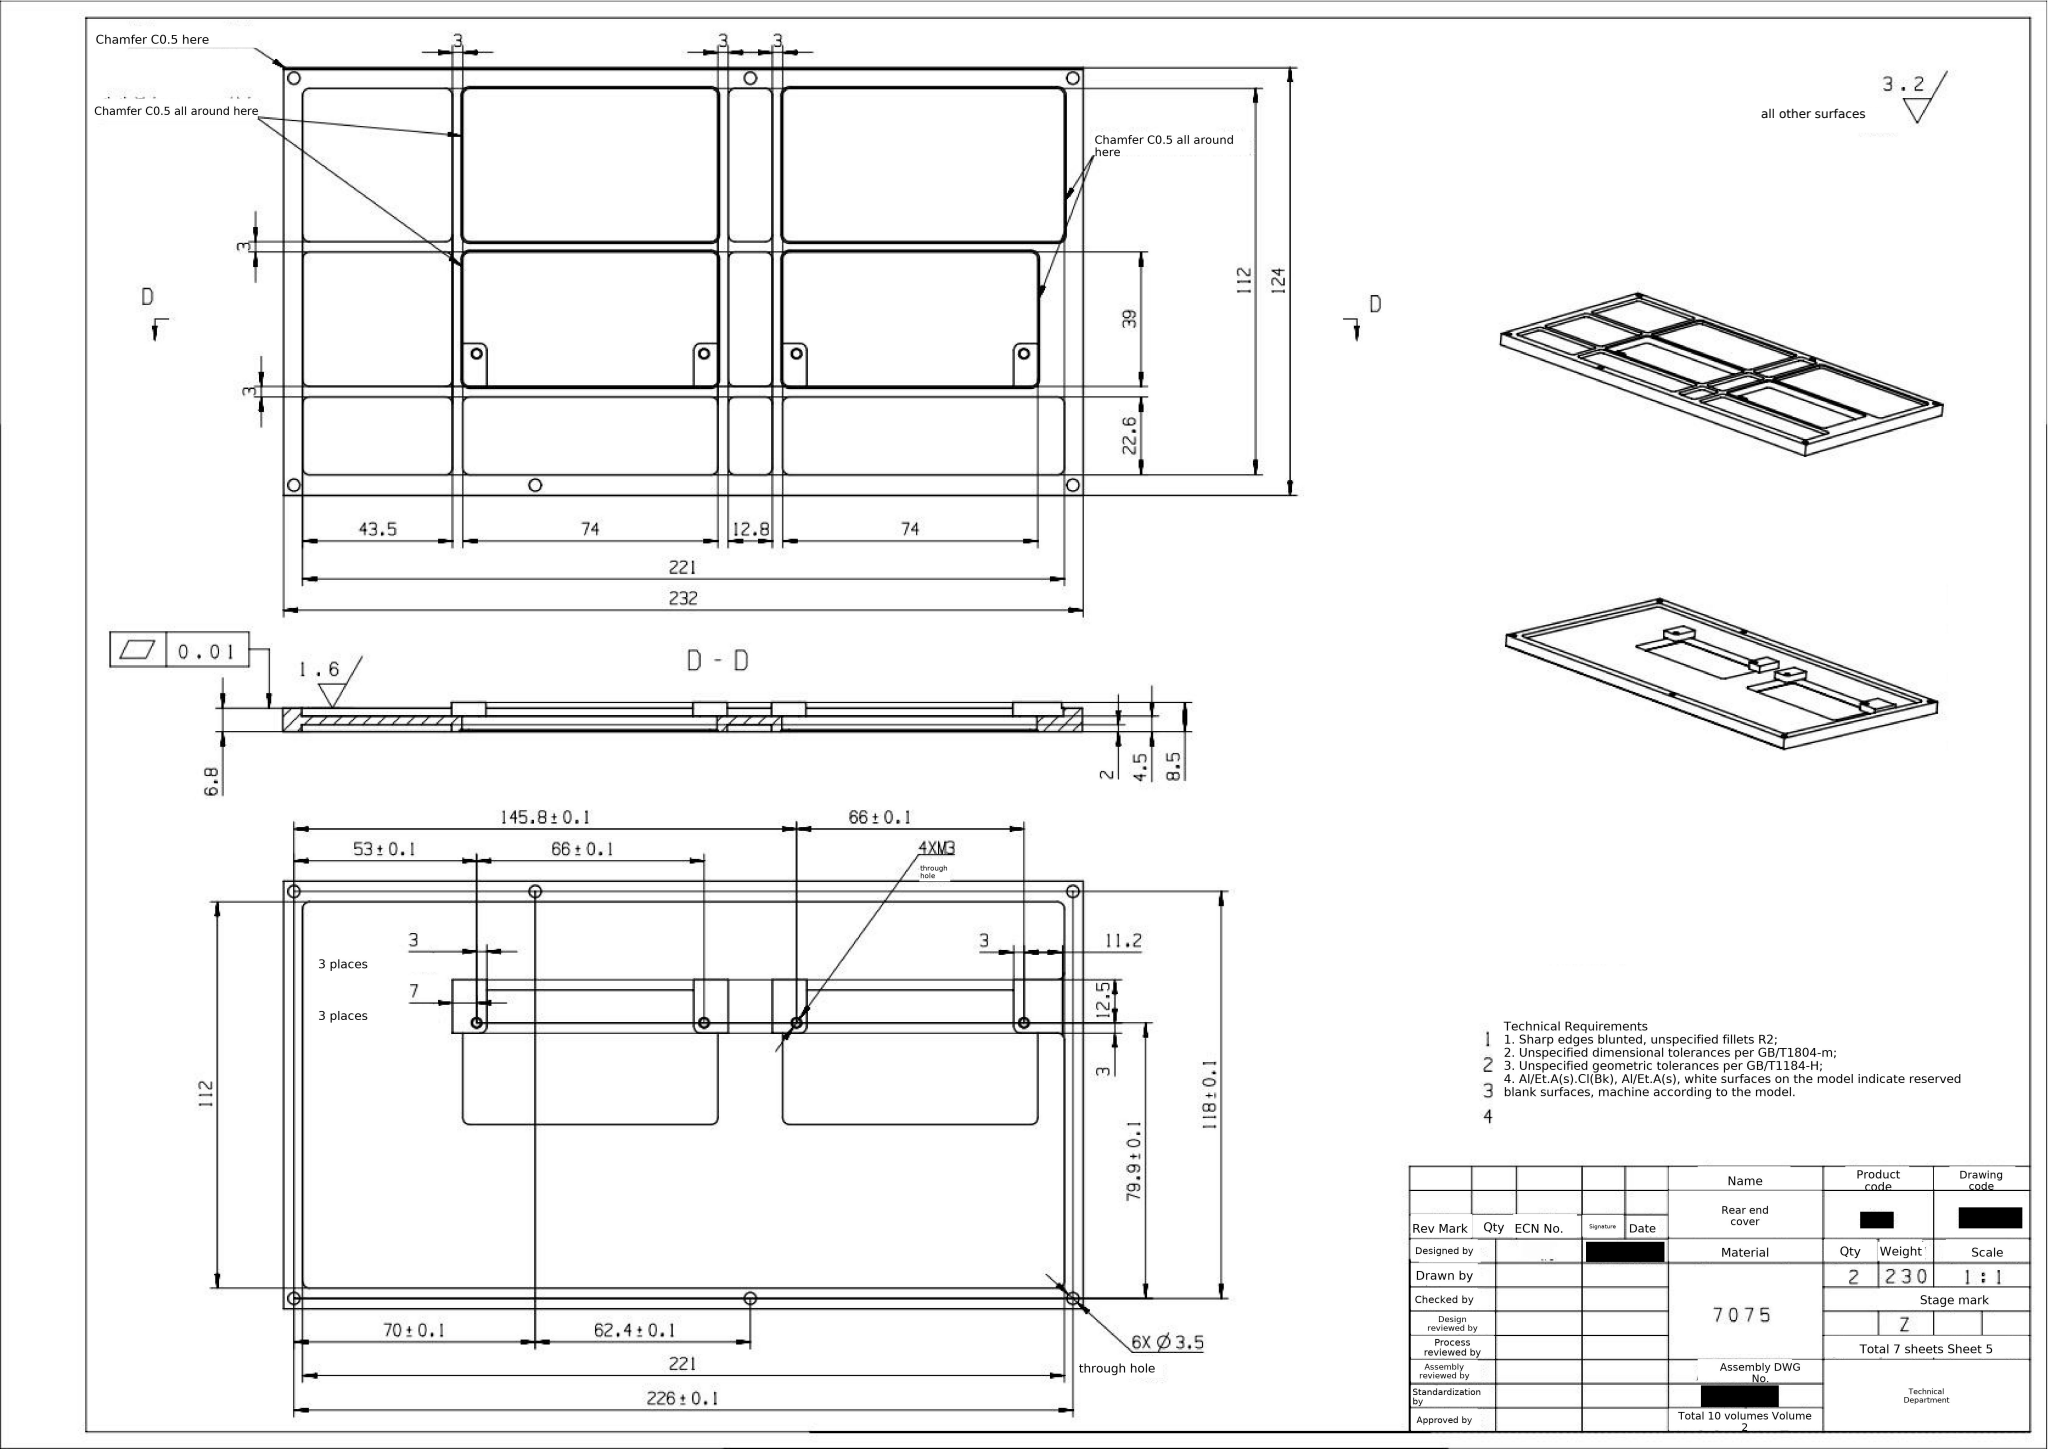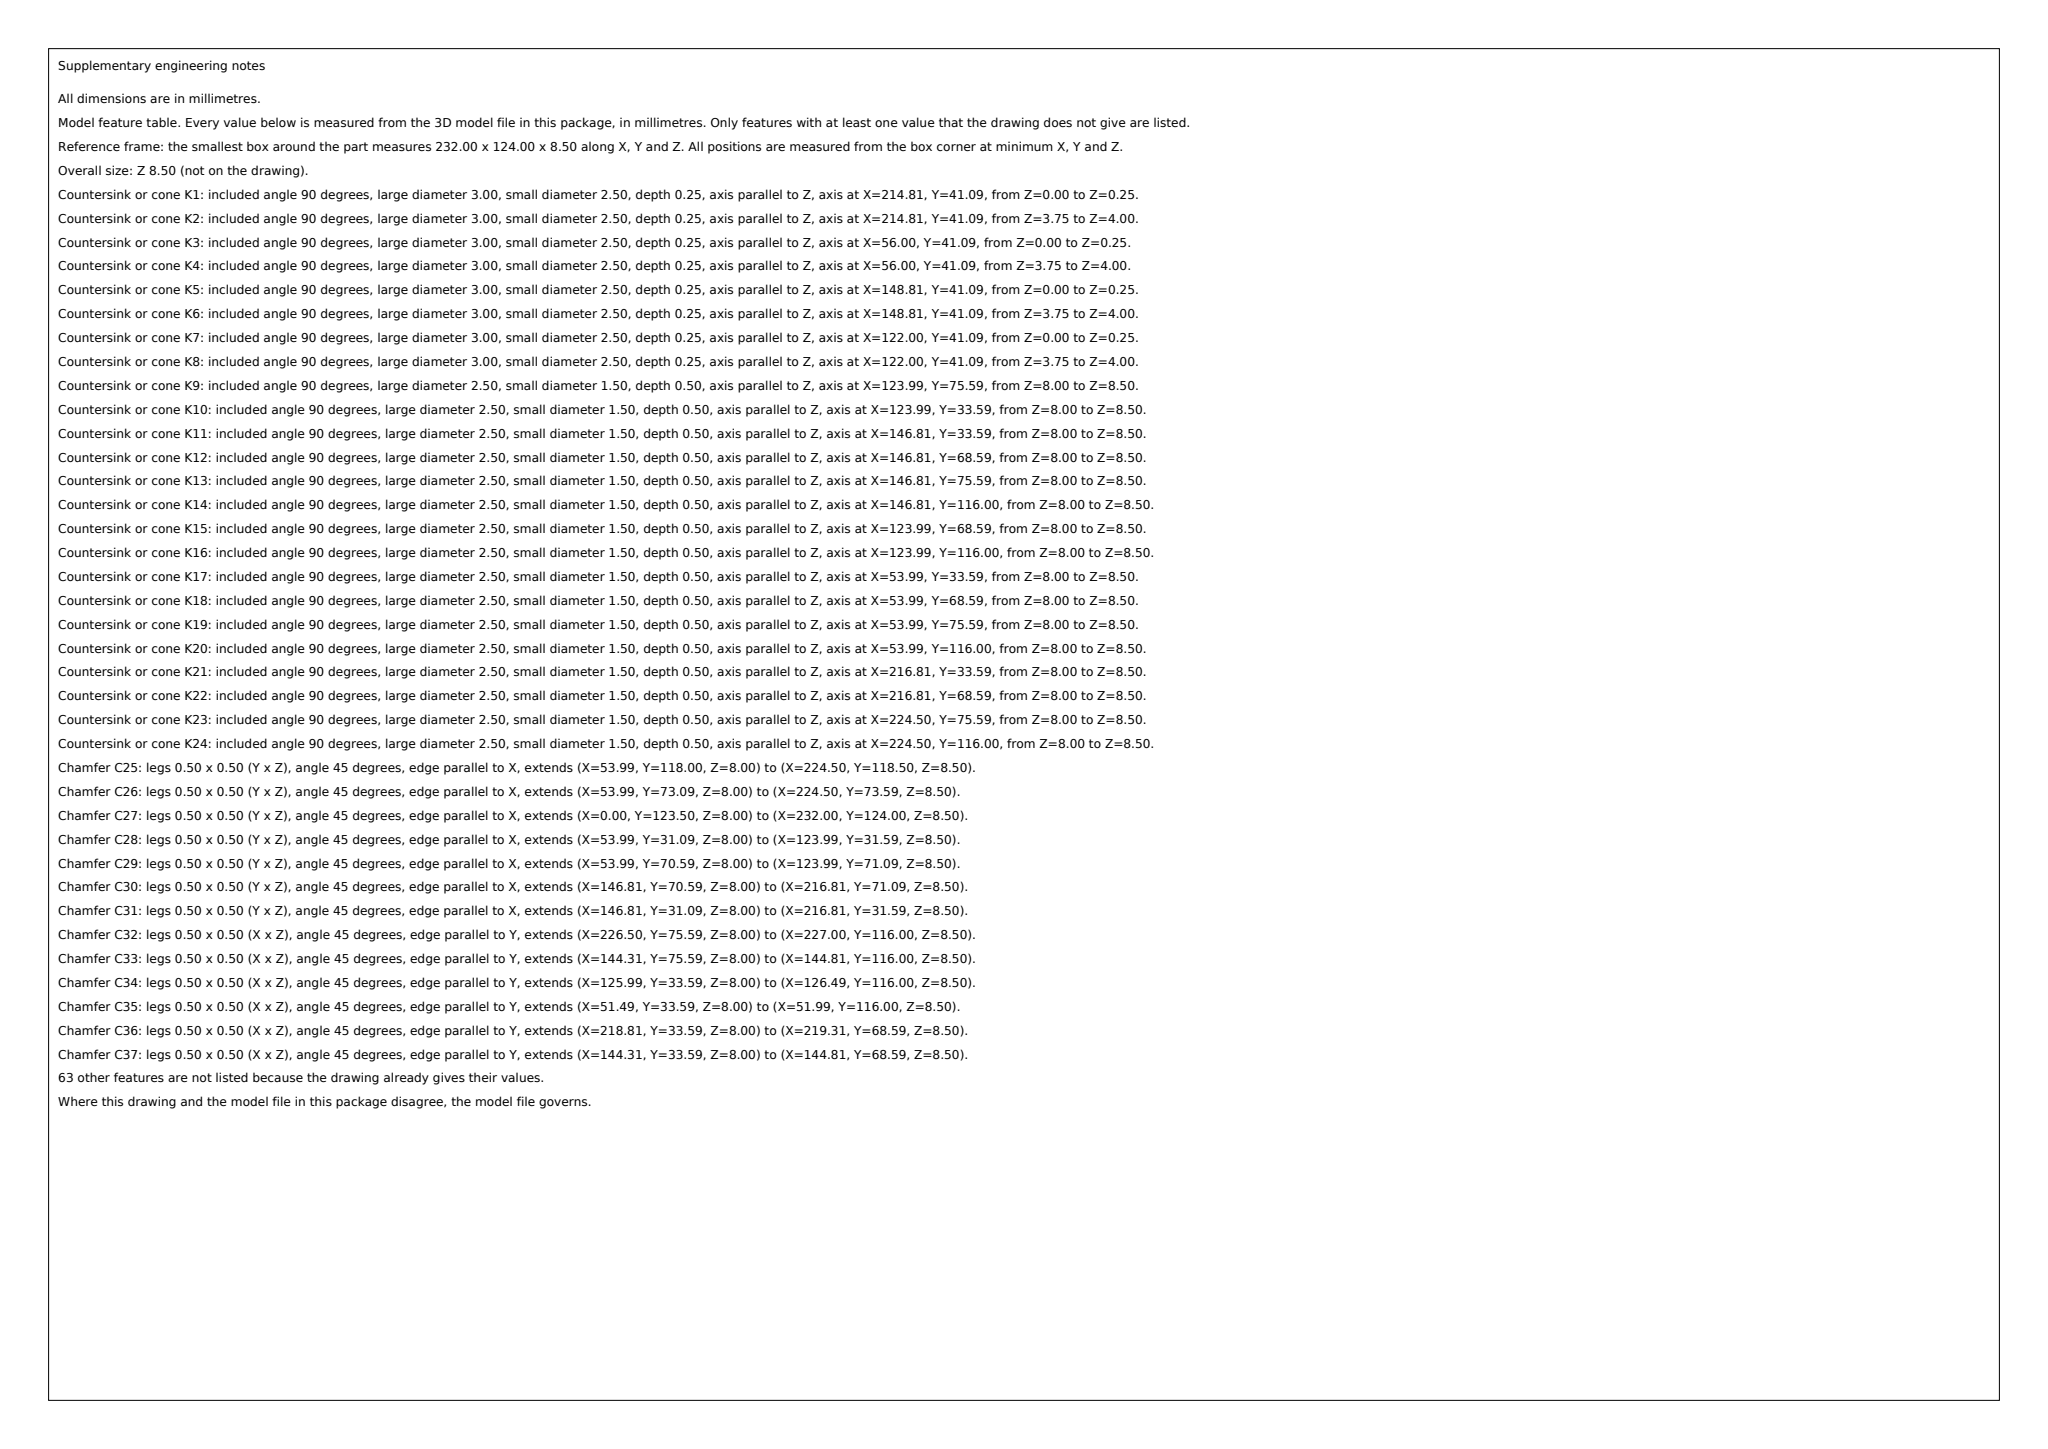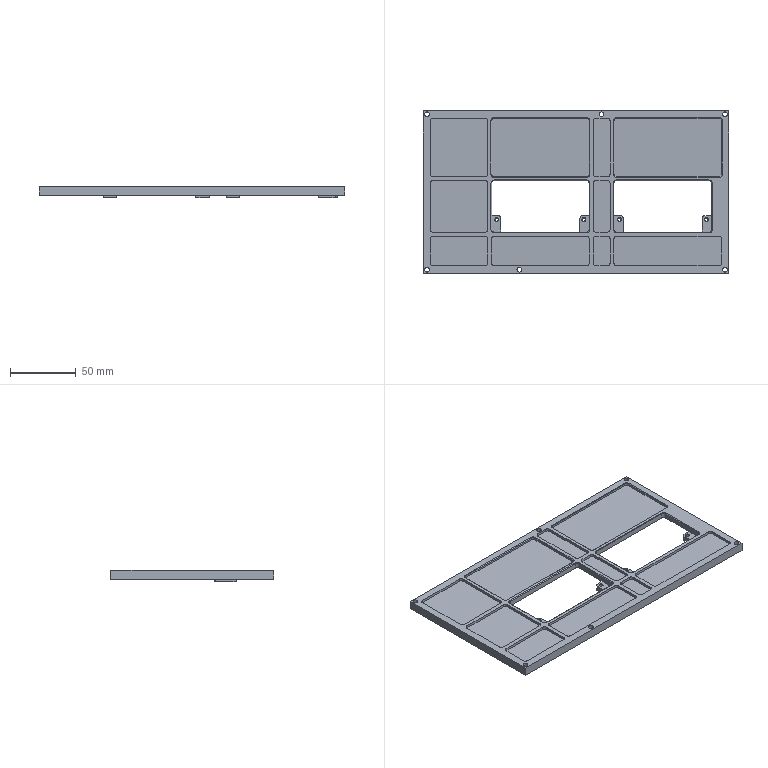Part | SolidWorks | mm | material 7075 | 1 solid | 221 faces | box 232 x 124 x 8.5 mm | volume 82154 mm3 | plane 111 | cylinder 78 | cone 32 | commonest cylinder face diameters 4 x58 3.5 x12 2.5 x8